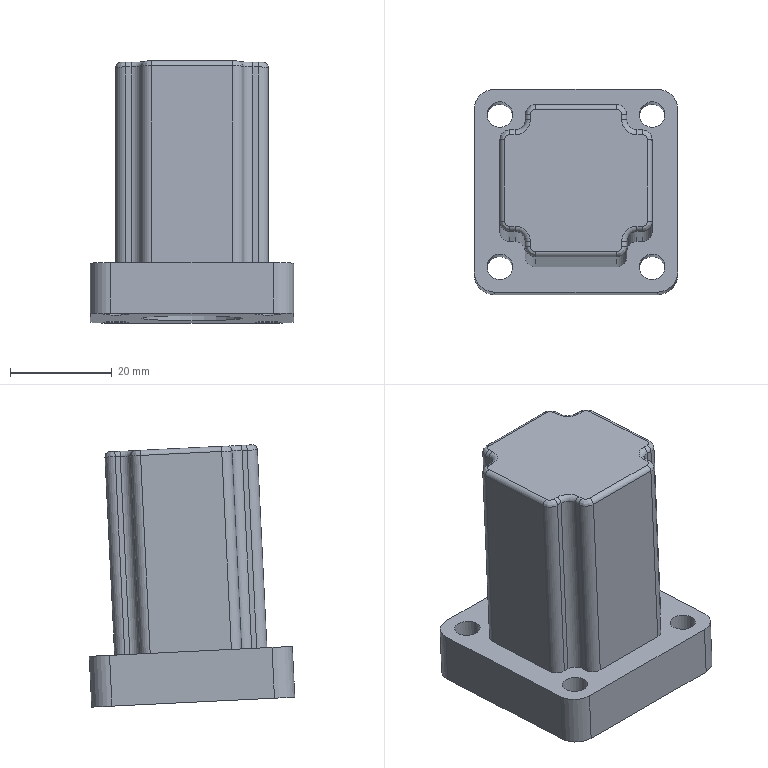Component | NX | CCJ-021 | 1 solid | 67 faces | volume 42676 mm3 | cylinder 34 | plane 21 | spline 8 | torus 4 | commonest cylinder face diameters 4 x12 2 x12 8 x4 5 x4 20 x1 10 x1